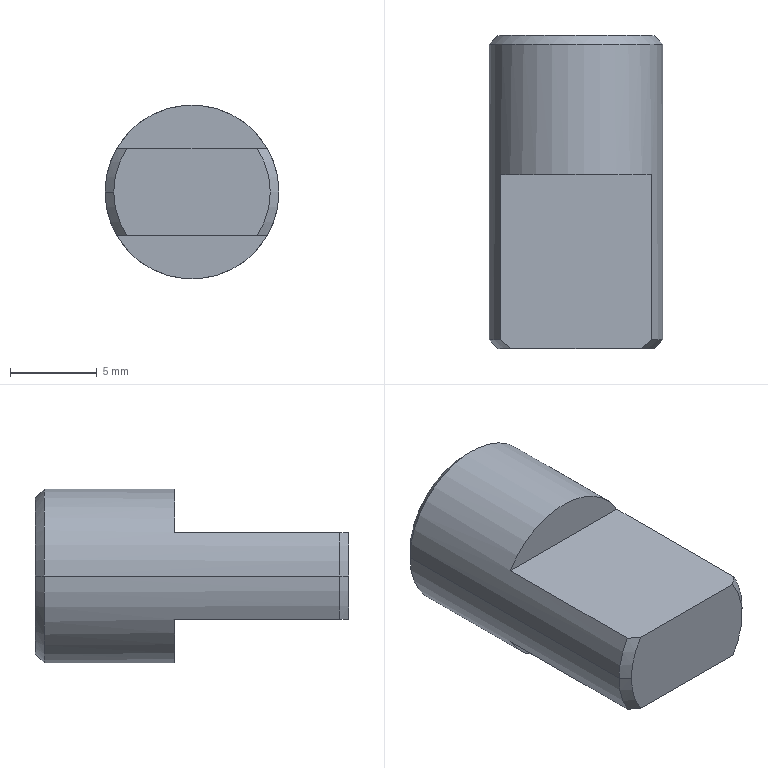Component | SolidWorks | MA060.03.03-09-11 | 1 solid | 17 faces | box 10 x 18 x 10 mm | volume 929 mm3 | cone 7 | plane 6 | cylinder 4 | commonest cylinder face diameters 4.2 x2 10 x2 | material Q235A
STEP:
#1=COLOUR_RGB('',0.7922,0.8196,0.9333);
#2=FILL_AREA_STYLE_COLOUR('',#1);
#3=FILL_AREA_STYLE('',(#2));
#4=SURFACE_STYLE_FILL_AREA(#3);
#5=SURFACE_SIDE_STYLE('',(#4));
#6=SURFACE_STYLE_USAGE(.BOTH.,#5);
#7=PRESENTATION_STYLE_ASSIGNMENT((#6));
#8=CARTESIAN_POINT('',(5.138,3.388,0.));
#9=VERTEX_POINT('',#8);
#10=CARTESIAN_POINT('',(5.492,3.388,0.));
#11=VERTEX_POINT('',#10);
#12=CARTESIAN_POINT('',(5.315,3.388,0.));
#13=DIRECTION('',(0.,1.,0.));
#14=DIRECTION('',(-1.,0.,0.));
#15=AXIS2_PLACEMENT_3D('',#12,#13,#14);
#16=CIRCLE('',#15,0.1772);
#17=EDGE_CURVE('',#9,#11,#16,.T.);
#18=ORIENTED_EDGE('',*,*,#17,.F.);
#19=CARTESIAN_POINT('',(5.118,3.368,0.));
#20=VERTEX_POINT('',#19);
#21=CARTESIAN_POINT('',(5.118,3.368,0.));
#22=DIRECTION('',(-0.7071,-0.7071,0.));
#23=VECTOR('',#22,39.37);
#24=LINE('',#21,#23);
#25=EDGE_CURVE('',#9,#20,#24,.T.);
#26=ORIENTED_EDGE('',*,*,#25,.T.);
#27=CARTESIAN_POINT('',(5.512,3.368,0.));
#28=VERTEX_POINT('',#27);
#29=CARTESIAN_POINT('',(5.315,3.368,0.));
#30=DIRECTION('',(-0.,-1.,-0.));
#31=DIRECTION('',(-1.,0.,0.));
#32=AXIS2_PLACEMENT_3D('',#29,#30,#31);
#33=CIRCLE('',#32,0.1969);
#34=EDGE_CURVE('',#28,#20,#33,.T.);
#35=ORIENTED_EDGE('',*,*,#34,.F.);
#36=CARTESIAN_POINT('',(5.512,3.368,0.));
#37=DIRECTION('',(0.7071,-0.7071,0.));
#38=VECTOR('',#37,39.37);
#39=LINE('',#36,#38);
#40=EDGE_CURVE('',#11,#28,#39,.T.);
#41=ORIENTED_EDGE('',*,*,#40,.F.);
#42=EDGE_LOOP('',(#18,#26,#35,#41));
#43=FACE_OUTER_BOUND('',#42,.T.);
#44=CARTESIAN_POINT('',(5.315,3.368,0.));
#45=DIRECTION('',(-0.,-1.,-0.));
#46=DIRECTION('',(1.,0.,0.));
#47=AXIS2_PLACEMENT_3D('',#44,#45,#46);
#48=CONICAL_SURFACE('',#47,0.1969,0.7854);
#49=ADVANCED_FACE('',(#43),#48,.T.);
#50=CARTESIAN_POINT('',(5.138,2.679,0.));
#51=VERTEX_POINT('',#50);
#52=CARTESIAN_POINT('',(5.168,2.679,-0.09843));
#53=VERTEX_POINT('',#52);
#54=CARTESIAN_POINT('',(5.315,2.679,0.));
#55=DIRECTION('',(0.,-1.,-0.));
#56=DIRECTION('',(1.,0.,0.));
#57=AXIS2_PLACEMENT_3D('',#54,#55,#56);
#58=CIRCLE('',#57,0.1772);
#59=EDGE_CURVE('',#51,#53,#58,.T.);
#60=ORIENTED_EDGE('',*,*,#59,.F.);
#61=CARTESIAN_POINT('',(5.118,2.699,0.));
#62=VERTEX_POINT('',#61);
#63=CARTESIAN_POINT('',(5.138,2.679,0.));
#64=DIRECTION('',(-0.7071,0.7071,0.));
#65=VECTOR('',#64,39.37);
#66=LINE('',#63,#65);
#67=EDGE_CURVE('',#51,#62,#66,.T.);
#68=ORIENTED_EDGE('',*,*,#67,.T.);
#69=CARTESIAN_POINT('',(5.144,2.699,-0.09843));
#70=VERTEX_POINT('',#69);
#71=CARTESIAN_POINT('',(5.315,2.699,0.));
#72=DIRECTION('',(0.,1.,0.));
#73=DIRECTION('',(1.,0.,-0.));
#74=AXIS2_PLACEMENT_3D('',#71,#72,#73);
#75=CIRCLE('',#74,0.1969);
#76=EDGE_CURVE('',#70,#62,#75,.T.);
#77=ORIENTED_EDGE('',*,*,#76,.F.);
#78=CARTESIAN_POINT('',(5.168,2.679,-0.09843));
#79=CARTESIAN_POINT('',(5.16,2.686,-0.09843));
#80=CARTESIAN_POINT('',(5.152,2.692,-0.09843));
#81=CARTESIAN_POINT('',(5.144,2.699,-0.09843));
#82=B_SPLINE_CURVE_WITH_KNOTS('',3,(#78,#79,#80,#81),.UNSPECIFIED.,.F.,.F.,(4,4),(0.,0.0007722),.UNSPECIFIED.);
#83=EDGE_CURVE('',#53,#70,#82,.T.);
#84=ORIENTED_EDGE('',*,*,#83,.F.);
#85=EDGE_LOOP('',(#60,#68,#77,#84));
#86=FACE_OUTER_BOUND('',#85,.T.);
#87=CARTESIAN_POINT('',(5.315,2.679,0.));
#88=DIRECTION('',(0.,1.,0.));
#89=DIRECTION('',(-1.,0.,0.));
#90=AXIS2_PLACEMENT_3D('',#87,#88,#89);
#91=CONICAL_SURFACE('',#90,0.1772,0.7854);
#92=ADVANCED_FACE('',(#86),#91,.T.);
#93=CARTESIAN_POINT('',(5.315,2.915,-0.08268));
#94=VERTEX_POINT('',#93);
#95=CARTESIAN_POINT('',(5.315,2.915,0.08268));
#96=VERTEX_POINT('',#95);
#97=CARTESIAN_POINT('',(5.315,2.915,0.));
#98=DIRECTION('',(-0.,1.,0.));
#99=DIRECTION('',(0.,0.,1.));
#100=AXIS2_PLACEMENT_3D('',#97,#98,#99);
#101=CIRCLE('',#100,0.08268);
#102=EDGE_CURVE('',#94,#96,#101,.T.);
#103=ORIENTED_EDGE('',*,*,#102,.F.);
#104=CARTESIAN_POINT('',(5.315,3.388,-0.08268));
#105=VERTEX_POINT('',#104);
#106=CARTESIAN_POINT('',(5.315,3.388,-0.08268));
#107=DIRECTION('',(-0.,1.,0.));
#108=VECTOR('',#107,39.37);
#109=LINE('',#106,#108);
#110=EDGE_CURVE('',#94,#105,#109,.T.);
#111=ORIENTED_EDGE('',*,*,#110,.T.);
#112=CARTESIAN_POINT('',(5.315,3.388,0.08268));
#113=VERTEX_POINT('',#112);
#114=CARTESIAN_POINT('',(5.315,3.388,0.));
#115=DIRECTION('',(-0.,1.,0.));
#116=DIRECTION('',(0.,0.,1.));
#117=AXIS2_PLACEMENT_3D('',#114,#115,#116);
#118=CIRCLE('',#117,0.08268);
#119=EDGE_CURVE('',#105,#113,#118,.T.);
#120=ORIENTED_EDGE('',*,*,#119,.T.);
#121=CARTESIAN_POINT('',(5.315,3.388,0.08268));
#122=DIRECTION('',(-0.,1.,0.));
#123=VECTOR('',#122,39.37);
#124=LINE('',#121,#123);
#125=EDGE_CURVE('',#96,#113,#124,.T.);
#126=ORIENTED_EDGE('',*,*,#125,.F.);
#127=EDGE_LOOP('',(#103,#111,#120,#126));
#128=FACE_OUTER_BOUND('',#127,.T.);
#129=CARTESIAN_POINT('',(5.315,3.388,0.));
#130=DIRECTION('',(-0.,1.,0.));
#131=DIRECTION('',(0.,0.,1.));
#132=AXIS2_PLACEMENT_3D('',#129,#130,#131);
#133=CYLINDRICAL_SURFACE('',#132,0.08268);
#134=ADVANCED_FACE('',(#128),#133,.F.);
#135=CARTESIAN_POINT('',(5.315,2.866,0.));
#136=VERTEX_POINT('',#135);
#137=CARTESIAN_POINT('',(5.315,2.915,0.08268));
#138=DIRECTION('',(-0.,0.515,0.8572));
#139=VECTOR('',#138,39.37);
#140=LINE('',#137,#139);
#141=EDGE_CURVE('',#136,#96,#140,.T.);
#142=ORIENTED_EDGE('',*,*,#141,.F.);
#143=CARTESIAN_POINT('',(5.315,2.915,-0.08268));
#144=DIRECTION('',(0.,0.515,-0.8572));
#145=VECTOR('',#144,39.37);
#146=LINE('',#143,#145);
#147=EDGE_CURVE('',#136,#94,#146,.T.);
#148=ORIENTED_EDGE('',*,*,#147,.T.);
#149=ORIENTED_EDGE('',*,*,#102,.T.);
#150=EDGE_LOOP('',(#142,#148,#149));
#151=FACE_OUTER_BOUND('',#150,.T.);
#152=CARTESIAN_POINT('',(5.315,2.915,0.));
#153=DIRECTION('',(-0.,1.,0.));
#154=DIRECTION('',(0.,0.,1.));
#155=AXIS2_PLACEMENT_3D('',#152,#153,#154);
#156=CONICAL_SURFACE('',#155,0.08268,1.03);
#157=ADVANCED_FACE('',(#151),#156,.F.);
#158=ORIENTED_EDGE('',*,*,#34,.T.);
#159=CARTESIAN_POINT('',(5.118,2.679,0.));
#160=DIRECTION('',(0.,-1.,-0.));
#161=VECTOR('',#160,39.37);
#162=LINE('',#159,#161);
#163=EDGE_CURVE('',#20,#62,#162,.T.);
#164=ORIENTED_EDGE('',*,*,#163,.T.);
#165=CARTESIAN_POINT('',(5.144,2.699,0.09843));
#166=VERTEX_POINT('',#165);
#167=CARTESIAN_POINT('',(5.315,2.699,0.));
#168=DIRECTION('',(0.,1.,0.));
#169=DIRECTION('',(1.,0.,-0.));
#170=AXIS2_PLACEMENT_3D('',#167,#168,#169);
#171=CIRCLE('',#170,0.1969);
#172=EDGE_CURVE('',#62,#166,#171,.T.);
#173=ORIENTED_EDGE('',*,*,#172,.T.);
#174=CARTESIAN_POINT('',(5.144,3.073,0.09843));
#175=VERTEX_POINT('',#174);
#176=CARTESIAN_POINT('',(5.144,3.073,0.09843));
#177=DIRECTION('',(0.,-1.,-0.));
#178=VECTOR('',#177,39.37);
#179=LINE('',#176,#178);
#180=EDGE_CURVE('',#175,#166,#179,.T.);
#181=ORIENTED_EDGE('',*,*,#180,.F.);
#182=CARTESIAN_POINT('',(5.485,3.073,0.09843));
#183=VERTEX_POINT('',#182);
#184=CARTESIAN_POINT('',(5.315,3.073,0.));
#185=DIRECTION('',(0.,1.,0.));
#186=DIRECTION('',(-1.,0.,0.));
#187=AXIS2_PLACEMENT_3D('',#184,#185,#186);
#188=CIRCLE('',#187,0.1969);
#189=EDGE_CURVE('',#175,#183,#188,.T.);
#190=ORIENTED_EDGE('',*,*,#189,.T.);
#191=CARTESIAN_POINT('',(5.485,2.699,0.09843));
#192=VERTEX_POINT('',#191);
#193=CARTESIAN_POINT('',(5.485,3.073,0.09843));
#194=DIRECTION('',(0.,-1.,-0.));
#195=VECTOR('',#194,39.37);
#196=LINE('',#193,#195);
#197=EDGE_CURVE('',#183,#192,#196,.T.);
#198=ORIENTED_EDGE('',*,*,#197,.T.);
#199=CARTESIAN_POINT('',(5.512,2.699,0.));
#200=VERTEX_POINT('',#199);
#201=CARTESIAN_POINT('',(5.315,2.699,0.));
#202=DIRECTION('',(0.,1.,0.));
#203=DIRECTION('',(1.,0.,-0.));
#204=AXIS2_PLACEMENT_3D('',#201,#202,#203);
#205=CIRCLE('',#204,0.1969);
#206=EDGE_CURVE('',#192,#200,#205,.T.);
#207=ORIENTED_EDGE('',*,*,#206,.T.);
#208=CARTESIAN_POINT('',(5.512,2.679,0.));
#209=DIRECTION('',(0.,-1.,-0.));
#210=VECTOR('',#209,39.37);
#211=LINE('',#208,#210);
#212=EDGE_CURVE('',#28,#200,#211,.T.);
#213=ORIENTED_EDGE('',*,*,#212,.F.);
#214=EDGE_LOOP('',(#158,#164,#173,#181,#190,#198,#207,#213));
#215=FACE_OUTER_BOUND('',#214,.T.);
#216=CARTESIAN_POINT('',(5.315,2.679,0.));
#217=DIRECTION('',(0.,-1.,-0.));
#218=DIRECTION('',(1.,0.,0.));
#219=AXIS2_PLACEMENT_3D('',#216,#217,#218);
#220=CYLINDRICAL_SURFACE('',#219,0.1969);
#221=ADVANCED_FACE('',(#215),#220,.T.);
#222=ORIENTED_EDGE('',*,*,#163,.F.);
#223=CARTESIAN_POINT('',(5.315,3.368,0.));
#224=DIRECTION('',(-0.,-1.,-0.));
#225=DIRECTION('',(-1.,0.,0.));
#226=AXIS2_PLACEMENT_3D('',#223,#224,#225);
#227=CIRCLE('',#226,0.1969);
#228=EDGE_CURVE('',#20,#28,#227,.T.);
#229=ORIENTED_EDGE('',*,*,#228,.T.);
#230=ORIENTED_EDGE('',*,*,#212,.T.);
#231=CARTESIAN_POINT('',(5.485,2.699,-0.09843));
#232=VERTEX_POINT('',#231);
#233=CARTESIAN_POINT('',(5.315,2.699,0.));
#234=DIRECTION('',(0.,1.,0.));
#235=DIRECTION('',(1.,0.,0.));
#236=AXIS2_PLACEMENT_3D('',#233,#234,#235);
#237=CIRCLE('',#236,0.1969);
#238=EDGE_CURVE('',#200,#232,#237,.T.);
#239=ORIENTED_EDGE('',*,*,#238,.T.);
#240=CARTESIAN_POINT('',(5.485,3.073,-0.09843));
#241=VERTEX_POINT('',#240);
#242=CARTESIAN_POINT('',(5.485,3.073,-0.09843));
#243=DIRECTION('',(0.,-1.,-0.));
#244=VECTOR('',#243,39.37);
#245=LINE('',#242,#244);
#246=EDGE_CURVE('',#241,#232,#245,.T.);
#247=ORIENTED_EDGE('',*,*,#246,.F.);
#248=CARTESIAN_POINT('',(5.144,3.073,-0.09843));
#249=VERTEX_POINT('',#248);
#250=CARTESIAN_POINT('',(5.315,3.073,0.));
#251=DIRECTION('',(0.,1.,0.));
#252=DIRECTION('',(-1.,0.,0.));
#253=AXIS2_PLACEMENT_3D('',#250,#251,#252);
#254=CIRCLE('',#253,0.1969);
#255=EDGE_CURVE('',#241,#249,#254,.T.);
#256=ORIENTED_EDGE('',*,*,#255,.T.);
#257=CARTESIAN_POINT('',(5.144,3.073,-0.09843));
#258=DIRECTION('',(0.,-1.,-0.));
#259=VECTOR('',#258,39.37);
#260=LINE('',#257,#259);
#261=EDGE_CURVE('',#249,#70,#260,.T.);
#262=ORIENTED_EDGE('',*,*,#261,.T.);
#263=ORIENTED_EDGE('',*,*,#76,.T.);
#264=EDGE_LOOP('',(#222,#229,#230,#239,#247,#256,#262,#263));
#265=FACE_OUTER_BOUND('',#264,.T.);
#266=CARTESIAN_POINT('',(5.315,2.679,0.));
#267=DIRECTION('',(0.,-1.,-0.));
#268=DIRECTION('',(1.,0.,0.));
#269=AXIS2_PLACEMENT_3D('',#266,#267,#268);
#270=CYLINDRICAL_SURFACE('',#269,0.1969);
#271=ADVANCED_FACE('',(#265),#270,.T.);
#272=CARTESIAN_POINT('',(5.462,2.679,0.09843));
#273=VERTEX_POINT('',#272);
#274=CARTESIAN_POINT('',(5.168,2.679,0.09843));
#275=VERTEX_POINT('',#274);
#276=CARTESIAN_POINT('',(5.485,2.679,0.09843));
#277=DIRECTION('',(-1.,-0.,-0.));
#278=VECTOR('',#277,39.37);
#279=LINE('',#276,#278);
#280=EDGE_CURVE('',#273,#275,#279,.T.);
#281=ORIENTED_EDGE('',*,*,#280,.T.);
#282=CARTESIAN_POINT('',(5.315,2.679,0.));
#283=DIRECTION('',(0.,-1.,-0.));
#284=DIRECTION('',(1.,0.,0.));
#285=AXIS2_PLACEMENT_3D('',#282,#283,#284);
#286=CIRCLE('',#285,0.1772);
#287=EDGE_CURVE('',#275,#51,#286,.T.);
#288=ORIENTED_EDGE('',*,*,#287,.T.);
#289=ORIENTED_EDGE('',*,*,#59,.T.);
#290=CARTESIAN_POINT('',(5.462,2.679,-0.09843));
#291=VERTEX_POINT('',#290);
#292=CARTESIAN_POINT('',(5.485,2.679,-0.09843));
#293=DIRECTION('',(1.,0.,-0.));
#294=VECTOR('',#293,39.37);
#295=LINE('',#292,#294);
#296=EDGE_CURVE('',#53,#291,#295,.T.);
#297=ORIENTED_EDGE('',*,*,#296,.T.);
#298=CARTESIAN_POINT('',(5.315,2.679,0.));
#299=DIRECTION('',(0.,-1.,-0.));
#300=DIRECTION('',(1.,0.,0.));
#301=AXIS2_PLACEMENT_3D('',#298,#299,#300);
#302=CIRCLE('',#301,0.1772);
#303=EDGE_CURVE('',#291,#273,#302,.T.);
#304=ORIENTED_EDGE('',*,*,#303,.T.);
#305=EDGE_LOOP('',(#281,#288,#289,#297,#304));
#306=FACE_OUTER_BOUND('',#305,.T.);
#307=CARTESIAN_POINT('',(5.512,2.679,0.));
#308=DIRECTION('',(0.,-1.,-0.));
#309=DIRECTION('',(1.,0.,0.));
#310=AXIS2_PLACEMENT_3D('',#307,#308,#309);
#311=PLANE('',#310);
#312=ADVANCED_FACE('',(#306),#311,.T.);
#313=CARTESIAN_POINT('',(5.315,3.388,0.));
#314=DIRECTION('',(0.,1.,0.));
#315=DIRECTION('',(-1.,0.,0.));
#316=AXIS2_PLACEMENT_3D('',#313,#314,#315);
#317=CIRCLE('',#316,0.1772);
#318=EDGE_CURVE('',#11,#9,#317,.T.);
#319=ORIENTED_EDGE('',*,*,#318,.T.);
#320=ORIENTED_EDGE('',*,*,#17,.T.);
#321=EDGE_LOOP('',(#319,#320));
#322=FACE_OUTER_BOUND('',#321,.T.);
#323=CARTESIAN_POINT('',(5.315,3.388,0.));
#324=DIRECTION('',(-0.,1.,0.));
#325=DIRECTION('',(0.,0.,1.));
#326=AXIS2_PLACEMENT_3D('',#323,#324,#325);
#327=CIRCLE('',#326,0.08268);
#328=EDGE_CURVE('',#113,#105,#327,.T.);
#329=ORIENTED_EDGE('',*,*,#328,.F.);
#330=ORIENTED_EDGE('',*,*,#119,.F.);
#331=EDGE_LOOP('',(#329,#330));
#332=FACE_BOUND('',#331,.T.);
#333=CARTESIAN_POINT('',(5.315,3.388,0.));
#334=DIRECTION('',(-0.,1.,0.));
#335=DIRECTION('',(-1.,0.,-0.));
#336=AXIS2_PLACEMENT_3D('',#333,#334,#335);
#337=PLANE('',#336);
#338=ADVANCED_FACE('',(#322,#332),#337,.T.);
#339=ORIENTED_EDGE('',*,*,#147,.F.);
#340=ORIENTED_EDGE('',*,*,#141,.T.);
#341=CARTESIAN_POINT('',(5.315,2.915,0.));
#342=DIRECTION('',(-0.,1.,0.));
#343=DIRECTION('',(0.,0.,1.));
#344=AXIS2_PLACEMENT_3D('',#341,#342,#343);
#345=CIRCLE('',#344,0.08268);
#346=EDGE_CURVE('',#96,#94,#345,.T.);
#347=ORIENTED_EDGE('',*,*,#346,.T.);
#348=EDGE_LOOP('',(#339,#340,#347));
#349=FACE_OUTER_BOUND('',#348,.T.);
#350=CARTESIAN_POINT('',(5.315,2.915,0.));
#351=DIRECTION('',(-0.,1.,0.));
#352=DIRECTION('',(0.,0.,1.));
#353=AXIS2_PLACEMENT_3D('',#350,#351,#352);
#354=CONICAL_SURFACE('',#353,0.08268,1.03);
#355=ADVANCED_FACE('',(#349),#354,.F.);
#356=ORIENTED_EDGE('',*,*,#110,.F.);
#357=ORIENTED_EDGE('',*,*,#346,.F.);
#358=ORIENTED_EDGE('',*,*,#125,.T.);
#359=ORIENTED_EDGE('',*,*,#328,.T.);
#360=EDGE_LOOP('',(#356,#357,#358,#359));
#361=FACE_OUTER_BOUND('',#360,.T.);
#362=CARTESIAN_POINT('',(5.315,3.388,0.));
#363=DIRECTION('',(-0.,1.,0.));
#364=DIRECTION('',(0.,0.,1.));
#365=AXIS2_PLACEMENT_3D('',#362,#363,#364);
#366=CYLINDRICAL_SURFACE('',#365,0.08268);
#367=ADVANCED_FACE('',(#361),#366,.F.);
#368=ORIENTED_EDGE('',*,*,#180,.T.);
#369=CARTESIAN_POINT('',(5.144,2.699,0.09843));
#370=CARTESIAN_POINT('',(5.152,2.692,0.09843));
#371=CARTESIAN_POINT('',(5.16,2.686,0.09843));
#372=CARTESIAN_POINT('',(5.168,2.679,0.09843));
#373=B_SPLINE_CURVE_WITH_KNOTS('',3,(#369,#370,#371,#372),.UNSPECIFIED.,.F.,.F.,(4,4),(0.,0.0007722),.UNSPECIFIED.);
#374=EDGE_CURVE('',#166,#275,#373,.T.);
#375=ORIENTED_EDGE('',*,*,#374,.T.);
#376=ORIENTED_EDGE('',*,*,#280,.F.);
#377=CARTESIAN_POINT('',(5.462,2.679,0.09843));
#378=CARTESIAN_POINT('',(5.47,2.686,0.09843));
#379=CARTESIAN_POINT('',(5.478,2.692,0.09843));
#380=CARTESIAN_POINT('',(5.485,2.699,0.09843));
#381=B_SPLINE_CURVE_WITH_KNOTS('',3,(#377,#378,#379,#380),.UNSPECIFIED.,.F.,.F.,(4,4),(0.,0.0007722),.UNSPECIFIED.);
#382=EDGE_CURVE('',#273,#192,#381,.T.);
#383=ORIENTED_EDGE('',*,*,#382,.T.);
#384=ORIENTED_EDGE('',*,*,#197,.F.);
#385=CARTESIAN_POINT('',(5.485,3.073,0.09843));
#386=DIRECTION('',(-1.,-0.,-0.));
#387=VECTOR('',#386,39.37);
#388=LINE('',#385,#387);
#389=EDGE_CURVE('',#183,#175,#388,.T.);
#390=ORIENTED_EDGE('',*,*,#389,.T.);
#391=EDGE_LOOP('',(#368,#375,#376,#383,#384,#390));
#392=FACE_OUTER_BOUND('',#391,.T.);
#393=CARTESIAN_POINT('',(5.485,3.073,0.09843));
#394=DIRECTION('',(-0.,-0.,1.));
#395=DIRECTION('',(0.,-1.,-0.));
#396=AXIS2_PLACEMENT_3D('',#393,#394,#395);
#397=PLANE('',#396);
#398=ADVANCED_FACE('',(#392),#397,.T.);
#399=ORIENTED_EDGE('',*,*,#189,.F.);
#400=ORIENTED_EDGE('',*,*,#389,.F.);
#401=EDGE_LOOP('',(#399,#400));
#402=FACE_OUTER_BOUND('',#401,.T.);
#403=CARTESIAN_POINT('',(5.315,3.073,0.));
#404=DIRECTION('',(-0.,1.,0.));
#405=DIRECTION('',(-1.,0.,-0.));
#406=AXIS2_PLACEMENT_3D('',#403,#404,#405);
#407=PLANE('',#406);
#408=ADVANCED_FACE('',(#402),#407,.F.);
#409=ORIENTED_EDGE('',*,*,#296,.F.);
#410=ORIENTED_EDGE('',*,*,#83,.T.);
#411=ORIENTED_EDGE('',*,*,#261,.F.);
#412=CARTESIAN_POINT('',(5.485,3.073,-0.09843));
#413=DIRECTION('',(1.,0.,-0.));
#414=VECTOR('',#413,39.37);
#415=LINE('',#412,#414);
#416=EDGE_CURVE('',#249,#241,#415,.T.);
#417=ORIENTED_EDGE('',*,*,#416,.T.);
#418=ORIENTED_EDGE('',*,*,#246,.T.);
#419=CARTESIAN_POINT('',(5.485,2.699,-0.09843));
#420=CARTESIAN_POINT('',(5.478,2.692,-0.09843));
#421=CARTESIAN_POINT('',(5.47,2.686,-0.09843));
#422=CARTESIAN_POINT('',(5.462,2.679,-0.09843));
#423=B_SPLINE_CURVE_WITH_KNOTS('',3,(#419,#420,#421,#422),.UNSPECIFIED.,.F.,.F.,(4,4),(0.,0.0007722),.UNSPECIFIED.);
#424=EDGE_CURVE('',#232,#291,#423,.T.);
#425=ORIENTED_EDGE('',*,*,#424,.T.);
#426=EDGE_LOOP('',(#409,#410,#411,#417,#418,#425));
#427=FACE_OUTER_BOUND('',#426,.T.);
#428=CARTESIAN_POINT('',(5.485,3.073,-0.09843));
#429=DIRECTION('',(-0.,0.,-1.));
#430=DIRECTION('',(1.,0.,-0.));
#431=AXIS2_PLACEMENT_3D('',#428,#429,#430);
#432=PLANE('',#431);
#433=ADVANCED_FACE('',(#427),#432,.T.);
#434=ORIENTED_EDGE('',*,*,#255,.F.);
#435=ORIENTED_EDGE('',*,*,#416,.F.);
#436=EDGE_LOOP('',(#434,#435));
#437=FACE_OUTER_BOUND('',#436,.T.);
#438=CARTESIAN_POINT('',(5.315,3.073,0.));
#439=DIRECTION('',(-0.,1.,0.));
#440=DIRECTION('',(-1.,0.,-0.));
#441=AXIS2_PLACEMENT_3D('',#438,#439,#440);
#442=PLANE('',#441);
#443=ADVANCED_FACE('',(#437),#442,.F.);
#444=ORIENTED_EDGE('',*,*,#67,.F.);
#445=ORIENTED_EDGE('',*,*,#287,.F.);
#446=ORIENTED_EDGE('',*,*,#374,.F.);
#447=ORIENTED_EDGE('',*,*,#172,.F.);
#448=EDGE_LOOP('',(#444,#445,#446,#447));
#449=FACE_OUTER_BOUND('',#448,.T.);
#450=CARTESIAN_POINT('',(5.315,2.679,0.));
#451=DIRECTION('',(0.,1.,0.));
#452=DIRECTION('',(-1.,0.,0.));
#453=AXIS2_PLACEMENT_3D('',#450,#451,#452);
#454=CONICAL_SURFACE('',#453,0.1772,0.7854);
#455=ADVANCED_FACE('',(#449),#454,.T.);
#456=ORIENTED_EDGE('',*,*,#424,.F.);
#457=ORIENTED_EDGE('',*,*,#238,.F.);
#458=ORIENTED_EDGE('',*,*,#206,.F.);
#459=ORIENTED_EDGE('',*,*,#382,.F.);
#460=ORIENTED_EDGE('',*,*,#303,.F.);
#461=EDGE_LOOP('',(#456,#457,#458,#459,#460));
#462=FACE_OUTER_BOUND('',#461,.T.);
#463=CARTESIAN_POINT('',(5.315,2.679,0.));
#464=DIRECTION('',(0.,1.,0.));
#465=DIRECTION('',(-1.,0.,0.));
#466=AXIS2_PLACEMENT_3D('',#463,#464,#465);
#467=CONICAL_SURFACE('',#466,0.1772,0.7854);
#468=ADVANCED_FACE('',(#462),#467,.T.);
#469=ORIENTED_EDGE('',*,*,#25,.F.);
#470=ORIENTED_EDGE('',*,*,#318,.F.);
#471=ORIENTED_EDGE('',*,*,#40,.T.);
#472=ORIENTED_EDGE('',*,*,#228,.F.);
#473=EDGE_LOOP('',(#469,#470,#471,#472));
#474=FACE_OUTER_BOUND('',#473,.T.);
#475=CARTESIAN_POINT('',(5.315,3.368,0.));
#476=DIRECTION('',(-0.,-1.,-0.));
#477=DIRECTION('',(1.,0.,0.));
#478=AXIS2_PLACEMENT_3D('',#475,#476,#477);
#479=CONICAL_SURFACE('',#478,0.1969,0.7854);
#480=ADVANCED_FACE('',(#474),#479,.T.);
#481=CLOSED_SHELL('',(#49,#92,#134,#157,#221,#271,#312,#338,#355,#367,#398,#408,#433,#443,#455,#468,#480));
#482=MANIFOLD_SOLID_BREP('',#481);
#483=STYLED_ITEM('',(#7),#482);
#484=PRESENTATION_LAYER_ASSIGNMENT('','',(#483));
#485=(LENGTH_UNIT()NAMED_UNIT(*)SI_UNIT($,.METRE.));
#486=LENGTH_MEASURE_WITH_UNIT(LENGTH_MEASURE(0.0254),#485);
#487=DIMENSIONAL_EXPONENTS(1.,0.,0.,0.,0.,0.,0.);
#488=(CONVERSION_BASED_UNIT('',#486)LENGTH_UNIT()NAMED_UNIT(#487));
#489=UNCERTAINTY_MEASURE_WITH_UNIT(LENGTH_MEASURE(0.00001),#488,'','');
#490=(NAMED_UNIT(*)PLANE_ANGLE_UNIT()SI_UNIT($,.RADIAN.));
#491=(NAMED_UNIT(*)SI_UNIT($,.STERADIAN.)SOLID_ANGLE_UNIT());
#492=(GEOMETRIC_REPRESENTATION_CONTEXT(3)GLOBAL_UNCERTAINTY_ASSIGNED_CONTEXT((#489))GLOBAL_UNIT_ASSIGNED_CONTEXT((#488,#490,#491))REPRESENTATION_CONTEXT('',''));
#493=MECHANICAL_DESIGN_GEOMETRIC_PRESENTATION_REPRESENTATION('',(#483),#492);
#494=CARTESIAN_POINT('',(0.,0.,0.));
#495=DIRECTION('',(0.,0.,1.));
#496=DIRECTION('',(1.,0.,0.));
#497=AXIS2_PLACEMENT_3D('',#494,#495,#496);
#498=(LENGTH_UNIT()NAMED_UNIT(*)SI_UNIT($,.METRE.));
#499=LENGTH_MEASURE_WITH_UNIT(LENGTH_MEASURE(0.0254),#498);
#500=DIMENSIONAL_EXPONENTS(1.,0.,0.,0.,0.,0.,0.);
#501=(CONVERSION_BASED_UNIT('',#499)LENGTH_UNIT()NAMED_UNIT(#500));
#502=UNCERTAINTY_MEASURE_WITH_UNIT(LENGTH_MEASURE(0.00001),#501,'','');
#503=(NAMED_UNIT(*)PLANE_ANGLE_UNIT()SI_UNIT($,.RADIAN.));
#504=(NAMED_UNIT(*)SI_UNIT($,.STERADIAN.)SOLID_ANGLE_UNIT());
#505=(GEOMETRIC_REPRESENTATION_CONTEXT(3)GLOBAL_UNCERTAINTY_ASSIGNED_CONTEXT((#502))GLOBAL_UNIT_ASSIGNED_CONTEXT((#501,#503,#504))REPRESENTATION_CONTEXT('',''));
#506=ADVANCED_BREP_SHAPE_REPRESENTATION('',(#482,#497),#505);